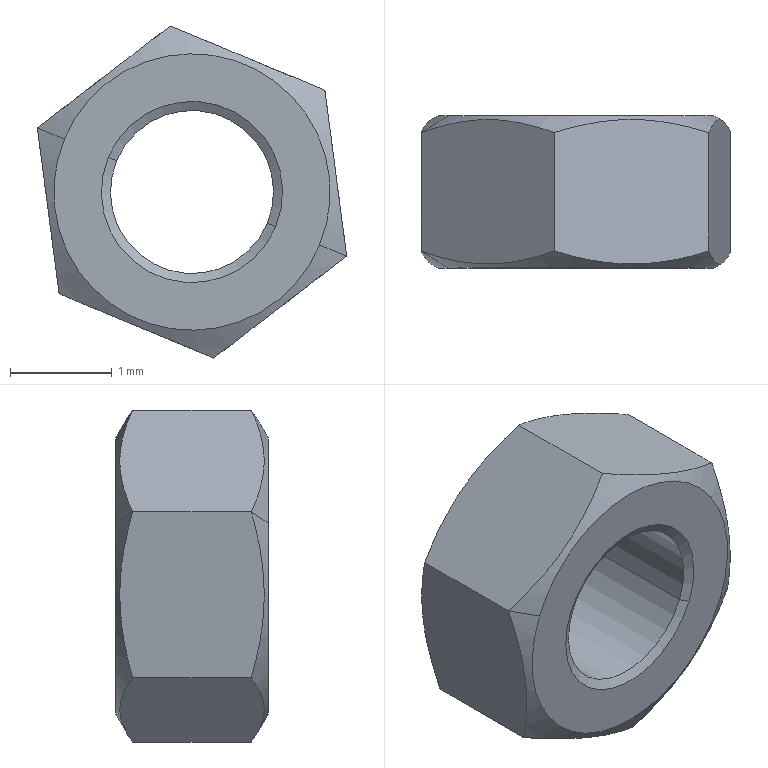Component | SolidWorks | Nut1-6 | 1 solid | 18 faces | box 3.03 x 1.49 x 3.26 mm | volume 7 mm3 | cone 8 | plane 8 | cylinder 2 | commonest cylinder face diameters 1.6 x2
STEP:
#1=COLOUR_RGB('',0.7922,0.8196,0.9333);
#2=FILL_AREA_STYLE_COLOUR('',#1);
#3=FILL_AREA_STYLE('',(#2));
#4=SURFACE_STYLE_FILL_AREA(#3);
#5=SURFACE_SIDE_STYLE('',(#4));
#6=SURFACE_STYLE_USAGE(.BOTH.,#5);
#7=PRESENTATION_STYLE_ASSIGNMENT((#6));
#8=CARTESIAN_POINT('',(0.6888,0.598,1.311));
#9=VERTEX_POINT('',#8);
#10=CARTESIAN_POINT('',(0.747,0.598,1.287));
#11=VERTEX_POINT('',#10);
#12=CARTESIAN_POINT('',(0.7179,0.598,1.299));
#13=DIRECTION('',(-0.,-1.,0.));
#14=DIRECTION('',(0.9237,0.,-0.383));
#15=AXIS2_PLACEMENT_3D('',#12,#13,#14);
#16=CIRCLE('',#15,0.0315);
#17=EDGE_CURVE('',#9,#11,#16,.T.);
#18=ORIENTED_EDGE('',*,*,#17,.F.);
#19=CARTESIAN_POINT('',(0.6856,0.596,1.313));
#20=VERTEX_POINT('',#19);
#21=CARTESIAN_POINT('',(0.6888,0.598,1.311));
#22=DIRECTION('',(-0.8,-0.5,0.3317));
#23=VECTOR('',#22,39.37);
#24=LINE('',#21,#23);
#25=EDGE_CURVE('',#9,#20,#24,.T.);
#26=ORIENTED_EDGE('',*,*,#25,.T.);
#27=CARTESIAN_POINT('',(0.7502,0.596,1.286));
#28=VERTEX_POINT('',#27);
#29=CARTESIAN_POINT('',(0.7179,0.596,1.299));
#30=DIRECTION('',(0.,1.,-0.));
#31=DIRECTION('',(0.9237,0.,-0.383));
#32=AXIS2_PLACEMENT_3D('',#29,#30,#31);
#33=CIRCLE('',#32,0.035);
#34=EDGE_CURVE('',#28,#20,#33,.T.);
#35=ORIENTED_EDGE('',*,*,#34,.F.);
#36=CARTESIAN_POINT('',(0.747,0.598,1.287));
#37=DIRECTION('',(0.8,-0.5,-0.3317));
#38=VECTOR('',#37,39.37);
#39=LINE('',#36,#38);
#40=EDGE_CURVE('',#11,#28,#39,.T.);
#41=ORIENTED_EDGE('',*,*,#40,.F.);
#42=EDGE_LOOP('',(#18,#26,#35,#41));
#43=FACE_OUTER_BOUND('',#42,.T.);
#44=CARTESIAN_POINT('',(0.7179,0.598,1.299));
#45=DIRECTION('',(-0.,-1.,0.));
#46=DIRECTION('',(0.9237,0.,-0.383));
#47=AXIS2_PLACEMENT_3D('',#44,#45,#46);
#48=CONICAL_SURFACE('',#47,0.0315,1.047);
#49=ADVANCED_FACE('',(#43),#48,.F.);
#50=CARTESIAN_POINT('',(0.747,0.6513,1.287));
#51=VERTEX_POINT('',#50);
#52=CARTESIAN_POINT('',(0.6888,0.6513,1.311));
#53=VERTEX_POINT('',#52);
#54=CARTESIAN_POINT('',(0.7179,0.6513,1.299));
#55=DIRECTION('',(0.,1.,-0.));
#56=DIRECTION('',(0.9237,0.,-0.383));
#57=AXIS2_PLACEMENT_3D('',#54,#55,#56);
#58=CIRCLE('',#57,0.0315);
#59=EDGE_CURVE('',#51,#53,#58,.T.);
#60=ORIENTED_EDGE('',*,*,#59,.F.);
#61=CARTESIAN_POINT('',(0.7489,0.6548,1.286));
#62=VERTEX_POINT('',#61);
#63=CARTESIAN_POINT('',(0.7489,0.6548,1.286));
#64=DIRECTION('',(0.4619,0.866,-0.1915));
#65=VECTOR('',#64,39.37);
#66=LINE('',#63,#65);
#67=EDGE_CURVE('',#51,#62,#66,.T.);
#68=ORIENTED_EDGE('',*,*,#67,.T.);
#69=CARTESIAN_POINT('',(0.6869,0.6548,1.312));
#70=VERTEX_POINT('',#69);
#71=CARTESIAN_POINT('',(0.7179,0.6548,1.299));
#72=DIRECTION('',(-0.,-1.,0.));
#73=DIRECTION('',(0.9237,0.,-0.383));
#74=AXIS2_PLACEMENT_3D('',#71,#72,#73);
#75=CIRCLE('',#74,0.03352);
#76=EDGE_CURVE('',#70,#62,#75,.T.);
#77=ORIENTED_EDGE('',*,*,#76,.F.);
#78=CARTESIAN_POINT('',(0.6869,0.6548,1.312));
#79=DIRECTION('',(-0.4619,0.866,0.1915));
#80=VECTOR('',#79,39.37);
#81=LINE('',#78,#80);
#82=EDGE_CURVE('',#53,#70,#81,.T.);
#83=ORIENTED_EDGE('',*,*,#82,.F.);
#84=EDGE_LOOP('',(#60,#68,#77,#83));
#85=FACE_OUTER_BOUND('',#84,.T.);
#86=CARTESIAN_POINT('',(0.7179,0.6548,1.299));
#87=DIRECTION('',(0.,1.,-0.));
#88=DIRECTION('',(-0.9237,0.,0.383));
#89=AXIS2_PLACEMENT_3D('',#86,#87,#88);
#90=CONICAL_SURFACE('',#89,0.03352,0.5236);
#91=ADVANCED_FACE('',(#85),#90,.F.);
#92=CARTESIAN_POINT('',(0.6686,0.596,1.32));
#93=VERTEX_POINT('',#92);
#94=CARTESIAN_POINT('',(0.7672,0.596,1.279));
#95=VERTEX_POINT('',#94);
#96=CARTESIAN_POINT('',(0.7179,0.596,1.299));
#97=DIRECTION('',(0.,1.,-0.));
#98=DIRECTION('',(-0.9237,0.,0.383));
#99=AXIS2_PLACEMENT_3D('',#96,#97,#98);
#100=CIRCLE('',#99,0.05337);
#101=EDGE_CURVE('',#93,#95,#100,.T.);
#102=ORIENTED_EDGE('',*,*,#101,.T.);
#103=CARTESIAN_POINT('',(0.7776,0.6025,1.274));
#104=VERTEX_POINT('',#103);
#105=CARTESIAN_POINT('',(0.7672,0.596,1.279));
#106=DIRECTION('',(0.8,0.5,-0.3317));
#107=VECTOR('',#106,39.37);
#108=LINE('',#105,#107);
#109=EDGE_CURVE('',#95,#104,#108,.T.);
#110=ORIENTED_EDGE('',*,*,#109,.T.);
#111=CARTESIAN_POINT('',(0.7692,0.6025,1.339));
#112=VERTEX_POINT('',#111);
#113=CARTESIAN_POINT('',(0.7776,0.6025,1.274));
#114=CARTESIAN_POINT('',(0.7763,0.5994,1.285));
#115=CARTESIAN_POINT('',(0.7749,0.5975,1.296));
#116=CARTESIAN_POINT('',(0.772,0.5975,1.317));
#117=CARTESIAN_POINT('',(0.7706,0.5994,1.328));
#118=CARTESIAN_POINT('',(0.7692,0.6025,1.339));
#119=B_SPLINE_CURVE_WITH_KNOTS('',3,(#113,#114,#115,#116,#117,#118),.UNSPECIFIED.,.F.,.F.,(4,2,4),(0.00000004,0.0008293,0.001659),.UNSPECIFIED.);
#120=EDGE_CURVE('',#104,#112,#119,.T.);
#121=ORIENTED_EDGE('',*,*,#120,.T.);
#122=CARTESIAN_POINT('',(0.7095,0.6025,1.363));
#123=VERTEX_POINT('',#122);
#124=CARTESIAN_POINT('',(0.7692,0.6025,1.339));
#125=CARTESIAN_POINT('',(0.7644,0.601,1.341));
#126=CARTESIAN_POINT('',(0.7595,0.5997,1.343));
#127=CARTESIAN_POINT('',(0.7495,0.598,1.347));
#128=CARTESIAN_POINT('',(0.7444,0.5975,1.349));
#129=CARTESIAN_POINT('',(0.7293,0.5975,1.355));
#130=CARTESIAN_POINT('',(0.7192,0.5995,1.359));
#131=CARTESIAN_POINT('',(0.7095,0.6025,1.363));
#132=B_SPLINE_CURVE_WITH_KNOTS('',3,(#124,#125,#126,#127,#128,#129,#130,#131),.UNSPECIFIED.,.F.,.F.,(4,2,2,4),(0.0006083,0.001023,0.001437,0.002266),.UNSPECIFIED.);
#133=EDGE_CURVE('',#112,#123,#132,.T.);
#134=ORIENTED_EDGE('',*,*,#133,.T.);
#135=CARTESIAN_POINT('',(0.6582,0.6025,1.324));
#136=VERTEX_POINT('',#135);
#137=CARTESIAN_POINT('',(0.7095,0.6025,1.363));
#138=CARTESIAN_POINT('',(0.7011,0.5994,1.357));
#139=CARTESIAN_POINT('',(0.6926,0.5975,1.35));
#140=CARTESIAN_POINT('',(0.6752,0.5975,1.337));
#141=CARTESIAN_POINT('',(0.6666,0.5994,1.33));
#142=CARTESIAN_POINT('',(0.6582,0.6025,1.324));
#143=B_SPLINE_CURVE_WITH_KNOTS('',3,(#137,#138,#139,#140,#141,#142),.UNSPECIFIED.,.F.,.F.,(4,2,4),(0.00000004,0.0008293,0.001659),.UNSPECIFIED.);
#144=EDGE_CURVE('',#123,#136,#143,.T.);
#145=ORIENTED_EDGE('',*,*,#144,.T.);
#146=CARTESIAN_POINT('',(0.6686,0.596,1.32));
#147=DIRECTION('',(-0.8,0.5,0.3317));
#148=VECTOR('',#147,39.37);
#149=LINE('',#146,#148);
#150=EDGE_CURVE('',#93,#136,#149,.T.);
#151=ORIENTED_EDGE('',*,*,#150,.F.);
#152=EDGE_LOOP('',(#102,#110,#121,#134,#145,#151));
#153=FACE_OUTER_BOUND('',#152,.T.);
#154=CARTESIAN_POINT('',(0.7179,0.596,1.299));
#155=DIRECTION('',(0.,1.,-0.));
#156=DIRECTION('',(-0.9237,0.,0.383));
#157=AXIS2_PLACEMENT_3D('',#154,#155,#156);
#158=CONICAL_SURFACE('',#157,0.05337,1.047);
#159=ADVANCED_FACE('',(#153),#158,.T.);
#160=CARTESIAN_POINT('',(0.6686,0.6548,1.32));
#161=VERTEX_POINT('',#160);
#162=CARTESIAN_POINT('',(0.7672,0.6548,1.279));
#163=VERTEX_POINT('',#162);
#164=CARTESIAN_POINT('',(0.7179,0.6548,1.299));
#165=DIRECTION('',(0.,1.,-0.));
#166=DIRECTION('',(-0.9237,0.,0.383));
#167=AXIS2_PLACEMENT_3D('',#164,#165,#166);
#168=CIRCLE('',#167,0.05337);
#169=EDGE_CURVE('',#161,#163,#168,.T.);
#170=ORIENTED_EDGE('',*,*,#169,.F.);
#171=CARTESIAN_POINT('',(0.6582,0.6482,1.324));
#172=VERTEX_POINT('',#171);
#173=CARTESIAN_POINT('',(0.6582,0.6482,1.324));
#174=DIRECTION('',(-0.8,-0.5,0.3317));
#175=VECTOR('',#174,39.37);
#176=LINE('',#173,#175);
#177=EDGE_CURVE('',#161,#172,#176,.T.);
#178=ORIENTED_EDGE('',*,*,#177,.T.);
#179=CARTESIAN_POINT('',(0.7095,0.6482,1.363));
#180=VERTEX_POINT('',#179);
#181=CARTESIAN_POINT('',(0.6582,0.6482,1.324));
#182=CARTESIAN_POINT('',(0.6666,0.6513,1.33));
#183=CARTESIAN_POINT('',(0.6751,0.6532,1.337));
#184=CARTESIAN_POINT('',(0.6925,0.6533,1.35));
#185=CARTESIAN_POINT('',(0.7011,0.6513,1.357));
#186=CARTESIAN_POINT('',(0.7095,0.6482,1.363));
#187=B_SPLINE_CURVE_WITH_KNOTS('',3,(#181,#182,#183,#184,#185,#186),.UNSPECIFIED.,.F.,.F.,(4,2,4),(0.00000004,0.0008293,0.001659),.UNSPECIFIED.);
#188=EDGE_CURVE('',#172,#180,#187,.T.);
#189=ORIENTED_EDGE('',*,*,#188,.T.);
#190=CARTESIAN_POINT('',(0.7692,0.6482,1.339));
#191=VERTEX_POINT('',#190);
#192=CARTESIAN_POINT('',(0.7095,0.6482,1.363));
#193=CARTESIAN_POINT('',(0.7192,0.6513,1.359));
#194=CARTESIAN_POINT('',(0.7293,0.6533,1.355));
#195=CARTESIAN_POINT('',(0.7444,0.6532,1.349));
#196=CARTESIAN_POINT('',(0.7495,0.6528,1.347));
#197=CARTESIAN_POINT('',(0.7595,0.651,1.343));
#198=CARTESIAN_POINT('',(0.7644,0.6498,1.341));
#199=CARTESIAN_POINT('',(0.7692,0.6482,1.339));
#200=B_SPLINE_CURVE_WITH_KNOTS('',3,(#192,#193,#194,#195,#196,#197,#198,#199),.UNSPECIFIED.,.F.,.F.,(4,2,2,4),(0.001459,0.00229,0.002705,0.003121),.UNSPECIFIED.);
#201=EDGE_CURVE('',#180,#191,#200,.T.);
#202=ORIENTED_EDGE('',*,*,#201,.T.);
#203=CARTESIAN_POINT('',(0.7776,0.6482,1.274));
#204=VERTEX_POINT('',#203);
#205=CARTESIAN_POINT('',(0.7692,0.6482,1.339));
#206=CARTESIAN_POINT('',(0.7706,0.6513,1.328));
#207=CARTESIAN_POINT('',(0.772,0.6532,1.317));
#208=CARTESIAN_POINT('',(0.7748,0.6533,1.296));
#209=CARTESIAN_POINT('',(0.7763,0.6513,1.285));
#210=CARTESIAN_POINT('',(0.7776,0.6482,1.274));
#211=B_SPLINE_CURVE_WITH_KNOTS('',3,(#205,#206,#207,#208,#209,#210),.UNSPECIFIED.,.F.,.F.,(4,2,4),(0.00000004,0.0008293,0.001659),.UNSPECIFIED.);
#212=EDGE_CURVE('',#191,#204,#211,.T.);
#213=ORIENTED_EDGE('',*,*,#212,.T.);
#214=CARTESIAN_POINT('',(0.7776,0.6482,1.274));
#215=DIRECTION('',(0.8,-0.5,-0.3317));
#216=VECTOR('',#215,39.37);
#217=LINE('',#214,#216);
#218=EDGE_CURVE('',#163,#204,#217,.T.);
#219=ORIENTED_EDGE('',*,*,#218,.F.);
#220=EDGE_LOOP('',(#170,#178,#189,#202,#213,#219));
#221=FACE_OUTER_BOUND('',#220,.T.);
#222=CARTESIAN_POINT('',(0.7179,0.6482,1.299));
#223=DIRECTION('',(-0.,-1.,0.));
#224=DIRECTION('',(0.9237,0.,-0.383));
#225=AXIS2_PLACEMENT_3D('',#222,#223,#224);
#226=CONICAL_SURFACE('',#225,0.06466,1.047);
#227=ADVANCED_FACE('',(#221),#226,.T.);
#228=ORIENTED_EDGE('',*,*,#59,.T.);
#229=CARTESIAN_POINT('',(0.6888,0.6548,1.311));
#230=DIRECTION('',(-0.,-1.,0.));
#231=VECTOR('',#230,39.37);
#232=LINE('',#229,#231);
#233=EDGE_CURVE('',#53,#9,#232,.T.);
#234=ORIENTED_EDGE('',*,*,#233,.T.);
#235=ORIENTED_EDGE('',*,*,#17,.T.);
#236=CARTESIAN_POINT('',(0.747,0.6548,1.287));
#237=DIRECTION('',(-0.,-1.,0.));
#238=VECTOR('',#237,39.37);
#239=LINE('',#236,#238);
#240=EDGE_CURVE('',#51,#11,#239,.T.);
#241=ORIENTED_EDGE('',*,*,#240,.F.);
#242=EDGE_LOOP('',(#228,#234,#235,#241));
#243=FACE_OUTER_BOUND('',#242,.T.);
#244=CARTESIAN_POINT('',(0.7179,0.6548,1.299));
#245=DIRECTION('',(-0.,-1.,0.));
#246=DIRECTION('',(0.9237,0.,-0.383));
#247=AXIS2_PLACEMENT_3D('',#244,#245,#246);
#248=CYLINDRICAL_SURFACE('',#247,0.0315);
#249=ADVANCED_FACE('',(#243),#248,.F.);
#250=CARTESIAN_POINT('',(0.7263,0.6025,1.235));
#251=VERTEX_POINT('',#250);
#252=CARTESIAN_POINT('',(0.7263,0.6025,1.235));
#253=CARTESIAN_POINT('',(0.7347,0.5994,1.242));
#254=CARTESIAN_POINT('',(0.7432,0.5975,1.248));
#255=CARTESIAN_POINT('',(0.7606,0.5975,1.261));
#256=CARTESIAN_POINT('',(0.7692,0.5994,1.268));
#257=CARTESIAN_POINT('',(0.7776,0.6025,1.274));
#258=B_SPLINE_CURVE_WITH_KNOTS('',3,(#252,#253,#254,#255,#256,#257),.UNSPECIFIED.,.F.,.F.,(4,2,4),(0.00000004,0.0008293,0.001659),.UNSPECIFIED.);
#259=EDGE_CURVE('',#251,#104,#258,.T.);
#260=ORIENTED_EDGE('',*,*,#259,.F.);
#261=CARTESIAN_POINT('',(0.7263,0.6482,1.235));
#262=VERTEX_POINT('',#261);
#263=CARTESIAN_POINT('',(0.7263,0.6548,1.235));
#264=DIRECTION('',(-0.,-1.,0.));
#265=VECTOR('',#264,39.37);
#266=LINE('',#263,#265);
#267=EDGE_CURVE('',#262,#251,#266,.T.);
#268=ORIENTED_EDGE('',*,*,#267,.F.);
#269=CARTESIAN_POINT('',(0.7776,0.6482,1.274));
#270=CARTESIAN_POINT('',(0.7692,0.6513,1.268));
#271=CARTESIAN_POINT('',(0.7607,0.6532,1.262));
#272=CARTESIAN_POINT('',(0.7433,0.6533,1.248));
#273=CARTESIAN_POINT('',(0.7347,0.6513,1.242));
#274=CARTESIAN_POINT('',(0.7263,0.6482,1.235));
#275=B_SPLINE_CURVE_WITH_KNOTS('',3,(#269,#270,#271,#272,#273,#274),.UNSPECIFIED.,.F.,.F.,(4,2,4),(0.00000004,0.0008293,0.001659),.UNSPECIFIED.);
#276=EDGE_CURVE('',#204,#262,#275,.T.);
#277=ORIENTED_EDGE('',*,*,#276,.F.);
#278=CARTESIAN_POINT('',(0.7776,0.6548,1.274));
#279=DIRECTION('',(-0.,-1.,0.));
#280=VECTOR('',#279,39.37);
#281=LINE('',#278,#280);
#282=EDGE_CURVE('',#204,#104,#281,.T.);
#283=ORIENTED_EDGE('',*,*,#282,.T.);
#284=EDGE_LOOP('',(#260,#268,#277,#283));
#285=FACE_OUTER_BOUND('',#284,.T.);
#286=CARTESIAN_POINT('',(0.7263,0.6548,1.235));
#287=DIRECTION('',(0.6084,-0.,-0.7936));
#288=DIRECTION('',(0.7936,-0.,0.6084));
#289=AXIS2_PLACEMENT_3D('',#286,#287,#288);
#290=PLANE('',#289);
#291=ADVANCED_FACE('',(#285),#290,.T.);
#292=CARTESIAN_POINT('',(0.6666,0.6025,1.26));
#293=VERTEX_POINT('',#292);
#294=CARTESIAN_POINT('',(0.6666,0.6025,1.26));
#295=CARTESIAN_POINT('',(0.6763,0.5995,1.256));
#296=CARTESIAN_POINT('',(0.6864,0.5975,1.252));
#297=CARTESIAN_POINT('',(0.7015,0.5975,1.245));
#298=CARTESIAN_POINT('',(0.7066,0.598,1.243));
#299=CARTESIAN_POINT('',(0.7166,0.5997,1.239));
#300=CARTESIAN_POINT('',(0.7215,0.601,1.237));
#301=CARTESIAN_POINT('',(0.7263,0.6025,1.235));
#302=B_SPLINE_CURVE_WITH_KNOTS('',3,(#294,#295,#296,#297,#298,#299,#300,#301),.UNSPECIFIED.,.F.,.F.,(4,2,2,4),(0.001459,0.00229,0.002705,0.003121),.UNSPECIFIED.);
#303=EDGE_CURVE('',#293,#251,#302,.T.);
#304=ORIENTED_EDGE('',*,*,#303,.F.);
#305=CARTESIAN_POINT('',(0.6666,0.6482,1.26));
#306=VERTEX_POINT('',#305);
#307=CARTESIAN_POINT('',(0.6666,0.6548,1.26));
#308=DIRECTION('',(-0.,-1.,0.));
#309=VECTOR('',#308,39.37);
#310=LINE('',#307,#309);
#311=EDGE_CURVE('',#306,#293,#310,.T.);
#312=ORIENTED_EDGE('',*,*,#311,.F.);
#313=CARTESIAN_POINT('',(0.7263,0.6482,1.235));
#314=CARTESIAN_POINT('',(0.7215,0.6498,1.237));
#315=CARTESIAN_POINT('',(0.7166,0.651,1.239));
#316=CARTESIAN_POINT('',(0.7066,0.6528,1.243));
#317=CARTESIAN_POINT('',(0.7015,0.6532,1.245));
#318=CARTESIAN_POINT('',(0.6864,0.6533,1.252));
#319=CARTESIAN_POINT('',(0.6763,0.6513,1.256));
#320=CARTESIAN_POINT('',(0.6666,0.6482,1.26));
#321=B_SPLINE_CURVE_WITH_KNOTS('',3,(#313,#314,#315,#316,#317,#318,#319,#320),.UNSPECIFIED.,.F.,.F.,(4,2,2,4),(0.0006083,0.001023,0.001437,0.002266),.UNSPECIFIED.);
#322=EDGE_CURVE('',#262,#306,#321,.T.);
#323=ORIENTED_EDGE('',*,*,#322,.F.);
#324=ORIENTED_EDGE('',*,*,#267,.T.);
#325=EDGE_LOOP('',(#304,#312,#323,#324));
#326=FACE_OUTER_BOUND('',#325,.T.);
#327=CARTESIAN_POINT('',(0.6666,0.6548,1.26));
#328=DIRECTION('',(-0.383,-0.,-0.9237));
#329=DIRECTION('',(0.,1.,-0.));
#330=AXIS2_PLACEMENT_3D('',#327,#328,#329);
#331=PLANE('',#330);
#332=ADVANCED_FACE('',(#326),#331,.T.);
#333=CARTESIAN_POINT('',(0.6582,0.6025,1.324));
#334=CARTESIAN_POINT('',(0.6596,0.5994,1.314));
#335=CARTESIAN_POINT('',(0.6609,0.5975,1.303));
#336=CARTESIAN_POINT('',(0.6638,0.5975,1.281));
#337=CARTESIAN_POINT('',(0.6652,0.5994,1.27));
#338=CARTESIAN_POINT('',(0.6666,0.6025,1.26));
#339=B_SPLINE_CURVE_WITH_KNOTS('',3,(#333,#334,#335,#336,#337,#338),.UNSPECIFIED.,.F.,.F.,(4,2,4),(0.00000004,0.0008293,0.001659),.UNSPECIFIED.);
#340=EDGE_CURVE('',#136,#293,#339,.T.);
#341=ORIENTED_EDGE('',*,*,#340,.F.);
#342=CARTESIAN_POINT('',(0.6582,0.6548,1.324));
#343=DIRECTION('',(-0.,-1.,0.));
#344=VECTOR('',#343,39.37);
#345=LINE('',#342,#344);
#346=EDGE_CURVE('',#172,#136,#345,.T.);
#347=ORIENTED_EDGE('',*,*,#346,.F.);
#348=CARTESIAN_POINT('',(0.6666,0.6482,1.26));
#349=CARTESIAN_POINT('',(0.6652,0.6513,1.27));
#350=CARTESIAN_POINT('',(0.6638,0.6532,1.281));
#351=CARTESIAN_POINT('',(0.661,0.6533,1.303));
#352=CARTESIAN_POINT('',(0.6596,0.6513,1.314));
#353=CARTESIAN_POINT('',(0.6582,0.6482,1.324));
#354=B_SPLINE_CURVE_WITH_KNOTS('',3,(#348,#349,#350,#351,#352,#353),.UNSPECIFIED.,.F.,.F.,(4,2,4),(0.00000004,0.0008293,0.001659),.UNSPECIFIED.);
#355=EDGE_CURVE('',#306,#172,#354,.T.);
#356=ORIENTED_EDGE('',*,*,#355,.F.);
#357=ORIENTED_EDGE('',*,*,#311,.T.);
#358=EDGE_LOOP('',(#341,#347,#356,#357));
#359=FACE_OUTER_BOUND('',#358,.T.);
#360=CARTESIAN_POINT('',(0.6582,0.6548,1.324));
#361=DIRECTION('',(-0.9915,0.,-0.1301));
#362=DIRECTION('',(0.1301,-0.,-0.9915));
#363=AXIS2_PLACEMENT_3D('',#360,#361,#362);
#364=PLANE('',#363);
#365=ADVANCED_FACE('',(#359),#364,.T.);
#366=ORIENTED_EDGE('',*,*,#144,.F.);
#367=CARTESIAN_POINT('',(0.7095,0.6548,1.363));
#368=DIRECTION('',(-0.,-1.,0.));
#369=VECTOR('',#368,39.37);
#370=LINE('',#367,#369);
#371=EDGE_CURVE('',#180,#123,#370,.T.);
#372=ORIENTED_EDGE('',*,*,#371,.F.);
#373=ORIENTED_EDGE('',*,*,#188,.F.);
#374=ORIENTED_EDGE('',*,*,#346,.T.);
#375=EDGE_LOOP('',(#366,#372,#373,#374));
#376=FACE_OUTER_BOUND('',#375,.T.);
#377=CARTESIAN_POINT('',(0.7095,0.6548,1.363));
#378=DIRECTION('',(-0.6084,0.,0.7936));
#379=DIRECTION('',(-0.7936,0.,-0.6084));
#380=AXIS2_PLACEMENT_3D('',#377,#378,#379);
#381=PLANE('',#380);
#382=ADVANCED_FACE('',(#376),#381,.T.);
#383=ORIENTED_EDGE('',*,*,#133,.F.);
#384=CARTESIAN_POINT('',(0.7692,0.6548,1.339));
#385=DIRECTION('',(-0.,-1.,0.));
#386=VECTOR('',#385,39.37);
#387=LINE('',#384,#386);
#388=EDGE_CURVE('',#191,#112,#387,.T.);
#389=ORIENTED_EDGE('',*,*,#388,.F.);
#390=ORIENTED_EDGE('',*,*,#201,.F.);
#391=ORIENTED_EDGE('',*,*,#371,.T.);
#392=EDGE_LOOP('',(#383,#389,#390,#391));
#393=FACE_OUTER_BOUND('',#392,.T.);
#394=CARTESIAN_POINT('',(0.7692,0.6548,1.339));
#395=DIRECTION('',(0.383,0.,0.9237));
#396=DIRECTION('',(-0.,-1.,0.));
#397=AXIS2_PLACEMENT_3D('',#394,#395,#396);
#398=PLANE('',#397);
#399=ADVANCED_FACE('',(#393),#398,.T.);
#400=ORIENTED_EDGE('',*,*,#120,.F.);
#401=ORIENTED_EDGE('',*,*,#282,.F.);
#402=ORIENTED_EDGE('',*,*,#212,.F.);
#403=ORIENTED_EDGE('',*,*,#388,.T.);
#404=EDGE_LOOP('',(#400,#401,#402,#403));
#405=FACE_OUTER_BOUND('',#404,.T.);
#406=CARTESIAN_POINT('',(0.7776,0.6548,1.274));
#407=DIRECTION('',(0.9915,-0.,0.1301));
#408=DIRECTION('',(-0.1301,0.,0.9915));
#409=AXIS2_PLACEMENT_3D('',#406,#407,#408);
#410=PLANE('',#409);
#411=ADVANCED_FACE('',(#405),#410,.T.);
#412=ORIENTED_EDGE('',*,*,#76,.T.);
#413=CARTESIAN_POINT('',(0.7179,0.6548,1.299));
#414=DIRECTION('',(-0.,-1.,0.));
#415=DIRECTION('',(0.9237,0.,-0.383));
#416=AXIS2_PLACEMENT_3D('',#413,#414,#415);
#417=CIRCLE('',#416,0.03352);
#418=EDGE_CURVE('',#62,#70,#417,.T.);
#419=ORIENTED_EDGE('',*,*,#418,.T.);
#420=EDGE_LOOP('',(#412,#419));
#421=FACE_BOUND('',#420,.T.);
#422=CARTESIAN_POINT('',(0.7179,0.6548,1.299));
#423=DIRECTION('',(0.,1.,-0.));
#424=DIRECTION('',(-0.9237,0.,0.383));
#425=AXIS2_PLACEMENT_3D('',#422,#423,#424);
#426=CIRCLE('',#425,0.05337);
#427=EDGE_CURVE('',#163,#161,#426,.T.);
#428=ORIENTED_EDGE('',*,*,#427,.T.);
#429=ORIENTED_EDGE('',*,*,#169,.T.);
#430=EDGE_LOOP('',(#428,#429));
#431=FACE_OUTER_BOUND('',#430,.T.);
#432=CARTESIAN_POINT('',(0.7776,0.6548,1.274));
#433=DIRECTION('',(-0.,-1.,0.));
#434=DIRECTION('',(0.9237,-0.,-0.383));
#435=AXIS2_PLACEMENT_3D('',#432,#433,#434);
#436=PLANE('',#435);
#437=ADVANCED_FACE('',(#421,#431),#436,.F.);
#438=ORIENTED_EDGE('',*,*,#34,.T.);
#439=CARTESIAN_POINT('',(0.7179,0.596,1.299));
#440=DIRECTION('',(0.,1.,-0.));
#441=DIRECTION('',(0.9237,0.,-0.383));
#442=AXIS2_PLACEMENT_3D('',#439,#440,#441);
#443=CIRCLE('',#442,0.035);
#444=EDGE_CURVE('',#20,#28,#443,.T.);
#445=ORIENTED_EDGE('',*,*,#444,.T.);
#446=EDGE_LOOP('',(#438,#445));
#447=FACE_BOUND('',#446,.T.);
#448=ORIENTED_EDGE('',*,*,#101,.F.);
#449=CARTESIAN_POINT('',(0.7179,0.596,1.299));
#450=DIRECTION('',(0.,1.,-0.));
#451=DIRECTION('',(-0.9237,0.,0.383));
#452=AXIS2_PLACEMENT_3D('',#449,#450,#451);
#453=CIRCLE('',#452,0.05337);
#454=EDGE_CURVE('',#95,#93,#453,.T.);
#455=ORIENTED_EDGE('',*,*,#454,.F.);
#456=EDGE_LOOP('',(#448,#455));
#457=FACE_OUTER_BOUND('',#456,.T.);
#458=CARTESIAN_POINT('',(0.7776,0.596,1.274));
#459=DIRECTION('',(-0.,-1.,0.));
#460=DIRECTION('',(0.9237,-0.,-0.383));
#461=AXIS2_PLACEMENT_3D('',#458,#459,#460);
#462=PLANE('',#461);
#463=ADVANCED_FACE('',(#447,#457),#462,.T.);
#464=ORIENTED_EDGE('',*,*,#233,.F.);
#465=CARTESIAN_POINT('',(0.7179,0.6513,1.299));
#466=DIRECTION('',(0.,1.,-0.));
#467=DIRECTION('',(0.9237,0.,-0.383));
#468=AXIS2_PLACEMENT_3D('',#465,#466,#467);
#469=CIRCLE('',#468,0.0315);
#470=EDGE_CURVE('',#53,#51,#469,.T.);
#471=ORIENTED_EDGE('',*,*,#470,.T.);
#472=ORIENTED_EDGE('',*,*,#240,.T.);
#473=CARTESIAN_POINT('',(0.7179,0.598,1.299));
#474=DIRECTION('',(-0.,-1.,0.));
#475=DIRECTION('',(0.9237,0.,-0.383));
#476=AXIS2_PLACEMENT_3D('',#473,#474,#475);
#477=CIRCLE('',#476,0.0315);
#478=EDGE_CURVE('',#11,#9,#477,.T.);
#479=ORIENTED_EDGE('',*,*,#478,.T.);
#480=EDGE_LOOP('',(#464,#471,#472,#479));
#481=FACE_OUTER_BOUND('',#480,.T.);
#482=CARTESIAN_POINT('',(0.7179,0.6548,1.299));
#483=DIRECTION('',(-0.,-1.,0.));
#484=DIRECTION('',(0.9237,0.,-0.383));
#485=AXIS2_PLACEMENT_3D('',#482,#483,#484);
#486=CYLINDRICAL_SURFACE('',#485,0.0315);
#487=ADVANCED_FACE('',(#481),#486,.F.);
#488=ORIENTED_EDGE('',*,*,#177,.F.);
#489=ORIENTED_EDGE('',*,*,#427,.F.);
#490=ORIENTED_EDGE('',*,*,#218,.T.);
#491=ORIENTED_EDGE('',*,*,#276,.T.);
#492=ORIENTED_EDGE('',*,*,#322,.T.);
#493=ORIENTED_EDGE('',*,*,#355,.T.);
#494=EDGE_LOOP('',(#488,#489,#490,#491,#492,#493));
#495=FACE_OUTER_BOUND('',#494,.T.);
#496=CARTESIAN_POINT('',(0.7179,0.6482,1.299));
#497=DIRECTION('',(-0.,-1.,0.));
#498=DIRECTION('',(0.9237,0.,-0.383));
#499=AXIS2_PLACEMENT_3D('',#496,#497,#498);
#500=CONICAL_SURFACE('',#499,0.06466,1.047);
#501=ADVANCED_FACE('',(#495),#500,.T.);
#502=ORIENTED_EDGE('',*,*,#109,.F.);
#503=ORIENTED_EDGE('',*,*,#454,.T.);
#504=ORIENTED_EDGE('',*,*,#150,.T.);
#505=ORIENTED_EDGE('',*,*,#340,.T.);
#506=ORIENTED_EDGE('',*,*,#303,.T.);
#507=ORIENTED_EDGE('',*,*,#259,.T.);
#508=EDGE_LOOP('',(#502,#503,#504,#505,#506,#507));
#509=FACE_OUTER_BOUND('',#508,.T.);
#510=CARTESIAN_POINT('',(0.7179,0.596,1.299));
#511=DIRECTION('',(0.,1.,-0.));
#512=DIRECTION('',(-0.9237,0.,0.383));
#513=AXIS2_PLACEMENT_3D('',#510,#511,#512);
#514=CONICAL_SURFACE('',#513,0.05337,1.047);
#515=ADVANCED_FACE('',(#509),#514,.T.);
#516=ORIENTED_EDGE('',*,*,#67,.F.);
#517=ORIENTED_EDGE('',*,*,#470,.F.);
#518=ORIENTED_EDGE('',*,*,#82,.T.);
#519=ORIENTED_EDGE('',*,*,#418,.F.);
#520=EDGE_LOOP('',(#516,#517,#518,#519));
#521=FACE_OUTER_BOUND('',#520,.T.);
#522=CARTESIAN_POINT('',(0.7179,0.6548,1.299));
#523=DIRECTION('',(0.,1.,-0.));
#524=DIRECTION('',(-0.9237,0.,0.383));
#525=AXIS2_PLACEMENT_3D('',#522,#523,#524);
#526=CONICAL_SURFACE('',#525,0.03352,0.5236);
#527=ADVANCED_FACE('',(#521),#526,.F.);
#528=ORIENTED_EDGE('',*,*,#25,.F.);
#529=ORIENTED_EDGE('',*,*,#478,.F.);
#530=ORIENTED_EDGE('',*,*,#40,.T.);
#531=ORIENTED_EDGE('',*,*,#444,.F.);
#532=EDGE_LOOP('',(#528,#529,#530,#531));
#533=FACE_OUTER_BOUND('',#532,.T.);
#534=CARTESIAN_POINT('',(0.7179,0.598,1.299));
#535=DIRECTION('',(-0.,-1.,0.));
#536=DIRECTION('',(0.9237,0.,-0.383));
#537=AXIS2_PLACEMENT_3D('',#534,#535,#536);
#538=CONICAL_SURFACE('',#537,0.0315,1.047);
#539=ADVANCED_FACE('',(#533),#538,.F.);
#540=CLOSED_SHELL('',(#49,#91,#159,#227,#249,#291,#332,#365,#382,#399,#411,#437,#463,#487,#501,#515,#527,#539));
#541=MANIFOLD_SOLID_BREP('',#540);
#542=STYLED_ITEM('',(#7),#541);
#543=PRESENTATION_LAYER_ASSIGNMENT('','',(#542));
#544=(LENGTH_UNIT()NAMED_UNIT(*)SI_UNIT($,.METRE.));
#545=LENGTH_MEASURE_WITH_UNIT(LENGTH_MEASURE(0.0254),#544);
#546=DIMENSIONAL_EXPONENTS(1.,0.,0.,0.,0.,0.,0.);
#547=(CONVERSION_BASED_UNIT('',#545)LENGTH_UNIT()NAMED_UNIT(#546));
#548=UNCERTAINTY_MEASURE_WITH_UNIT(LENGTH_MEASURE(0.00001),#547,'','');
#549=(NAMED_UNIT(*)PLANE_ANGLE_UNIT()SI_UNIT($,.RADIAN.));
#550=(NAMED_UNIT(*)SI_UNIT($,.STERADIAN.)SOLID_ANGLE_UNIT());
#551=(GEOMETRIC_REPRESENTATION_CONTEXT(3)GLOBAL_UNCERTAINTY_ASSIGNED_CONTEXT((#548))GLOBAL_UNIT_ASSIGNED_CONTEXT((#547,#549,#550))REPRESENTATION_CONTEXT('',''));
#552=MECHANICAL_DESIGN_GEOMETRIC_PRESENTATION_REPRESENTATION('',(#542),#551);
#553=CARTESIAN_POINT('',(0.,0.,0.));
#554=DIRECTION('',(0.,0.,1.));
#555=DIRECTION('',(1.,0.,0.));
#556=AXIS2_PLACEMENT_3D('',#553,#554,#555);
#557=(LENGTH_UNIT()NAMED_UNIT(*)SI_UNIT($,.METRE.));
#558=LENGTH_MEASURE_WITH_UNIT(LENGTH_MEASURE(0.0254),#557);
#559=DIMENSIONAL_EXPONENTS(1.,0.,0.,0.,0.,0.,0.);
#560=(CONVERSION_BASED_UNIT('',#558)LENGTH_UNIT()NAMED_UNIT(#559));
#561=UNCERTAINTY_MEASURE_WITH_UNIT(LENGTH_MEASURE(0.00001),#560,'','');
#562=(NAMED_UNIT(*)PLANE_ANGLE_UNIT()SI_UNIT($,.RADIAN.));
#563=(NAMED_UNIT(*)SI_UNIT($,.STERADIAN.)SOLID_ANGLE_UNIT());
#564=(GEOMETRIC_REPRESENTATION_CONTEXT(3)GLOBAL_UNCERTAINTY_ASSIGNED_CONTEXT((#561))GLOBAL_UNIT_ASSIGNED_CONTEXT((#560,#562,#563))REPRESENTATION_CONTEXT('',''));
#565=ADVANCED_BREP_SHAPE_REPRESENTATION('',(#541,#556),#564);